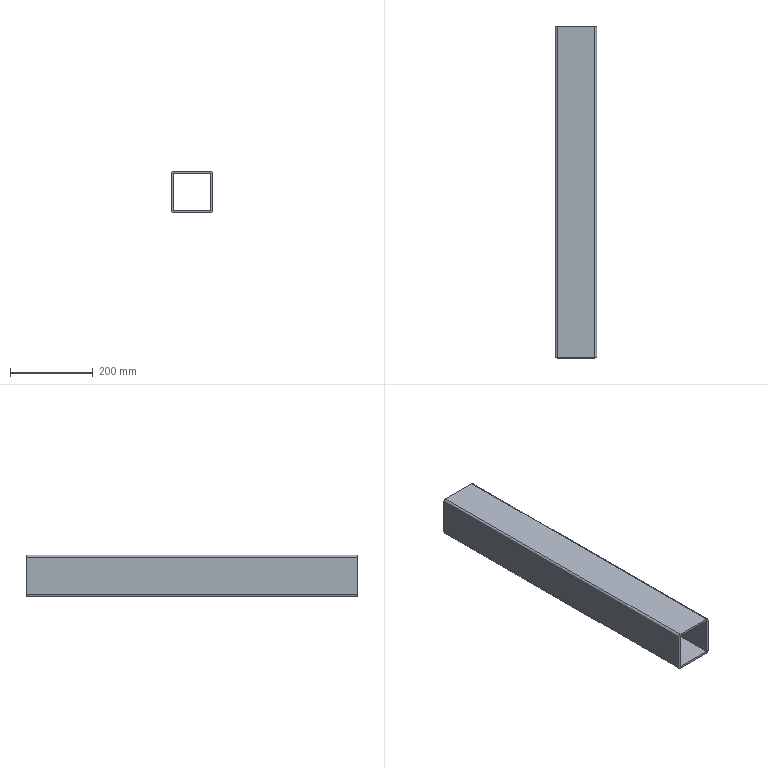Component | NX | TUBO | 1 solid | 14 faces | box 100 x 800 x 100 mm | volume 1502832 mm3 | plane 10 | cylinder 4 | commonest cylinder face diameters 10 x4
STEP:
#1=CARTESIAN_POINT('',(0.,0.,0.));
#2=DIRECTION('',(0.,0.,1.));
#3=DIRECTION('',(1.,0.,0.));
#4=AXIS2_PLACEMENT_3D('',#1,#2,#3);
#5=CARTESIAN_POINT('',(0.,65.2,795.));
#6=VERTEX_POINT('',#5);
#7=CARTESIAN_POINT('',(0.,65.2,705.));
#8=VERTEX_POINT('',#7);
#9=CARTESIAN_POINT('',(0.,65.2,795.));
#10=DIRECTION('',(0.,0.,-1.));
#11=VECTOR('',#10,1.);
#12=LINE('',#9,#11);
#13=CARTESIAN_POINT('',(0.,-734.8,795.));
#14=DIRECTION('',(1.,0.,0.));
#15=DIRECTION('',(0.,0.,-1.));
#16=AXIS2_PLACEMENT_3D('',#13,#14,#15);
#17=PLANE('',#16);
#18=CARTESIAN_POINT('',(0.,800.));
#19=DIRECTION('',(1.,0.));
#20=VECTOR('',#19,1.);
#21=LINE('',#18,#20);
#22=(GEOMETRIC_REPRESENTATION_CONTEXT(2)PARAMETRIC_REPRESENTATION_CONTEXT()REPRESENTATION_CONTEXT('',''));
#23=DEFINITIONAL_REPRESENTATION('',(#21),#22);
#24=PCURVE('',#17,#23);
#25=CARTESIAN_POINT('',(5.,65.2,705.));
#26=DIRECTION('',(0.,-1.,0.));
#27=DIRECTION('',(0.,0.,-1.));
#28=AXIS2_PLACEMENT_3D('',#25,#26,#27);
#29=PLANE('',#28);
#30=CARTESIAN_POINT('',(-90.,-5.));
#31=DIRECTION('',(1.,0.));
#32=VECTOR('',#31,1.);
#33=LINE('',#30,#32);
#34=(GEOMETRIC_REPRESENTATION_CONTEXT(2)PARAMETRIC_REPRESENTATION_CONTEXT()REPRESENTATION_CONTEXT('',''));
#35=DEFINITIONAL_REPRESENTATION('',(#33),#34);
#36=PCURVE('',#29,#35);
#37=SURFACE_CURVE('',#12,(#24,#36),.PCURVE_S1.);
#38=EDGE_CURVE('',#6,#8,#37,.T.);
#39=ORIENTED_EDGE('',*,*,#38,.T.);
#40=CARTESIAN_POINT('',(0.,-734.8,705.));
#41=VERTEX_POINT('',#40);
#42=CARTESIAN_POINT('',(0.,-734.8,705.));
#43=DIRECTION('',(0.,1.,0.));
#44=VECTOR('',#43,1.);
#45=LINE('',#42,#44);
#46=CARTESIAN_POINT('',(90.,0.));
#47=DIRECTION('',(0.,1.));
#48=VECTOR('',#47,1.);
#49=LINE('',#46,#48);
#50=(GEOMETRIC_REPRESENTATION_CONTEXT(2)PARAMETRIC_REPRESENTATION_CONTEXT()REPRESENTATION_CONTEXT('',''));
#51=DEFINITIONAL_REPRESENTATION('',(#49),#50);
#52=PCURVE('',#17,#51);
#53=CARTESIAN_POINT('',(5.,-734.8,705.));
#54=DIRECTION('',(0.,1.,0.));
#55=DIRECTION('',(0.,0.,1.));
#56=AXIS2_PLACEMENT_3D('',#53,#54,#55);
#57=CYLINDRICAL_SURFACE('',#56,5.);
#58=CARTESIAN_POINT('',(4.712,0.));
#59=DIRECTION('',(0.,1.));
#60=VECTOR('',#59,1.);
#61=LINE('',#58,#60);
#62=(GEOMETRIC_REPRESENTATION_CONTEXT(2)PARAMETRIC_REPRESENTATION_CONTEXT()REPRESENTATION_CONTEXT('',''));
#63=DEFINITIONAL_REPRESENTATION('',(#61),#62);
#64=PCURVE('',#57,#63);
#65=SURFACE_CURVE('',#45,(#52,#64),.PCURVE_S1.);
#66=EDGE_CURVE('',#41,#8,#65,.T.);
#67=ORIENTED_EDGE('',*,*,#66,.F.);
#68=CARTESIAN_POINT('',(0.,-734.8,795.));
#69=VERTEX_POINT('',#68);
#70=CARTESIAN_POINT('',(0.,-734.8,795.));
#71=DIRECTION('',(0.,0.,-1.));
#72=VECTOR('',#71,1.);
#73=LINE('',#70,#72);
#74=CARTESIAN_POINT('',(0.,0.));
#75=DIRECTION('',(1.,0.));
#76=VECTOR('',#75,1.);
#77=LINE('',#74,#76);
#78=(GEOMETRIC_REPRESENTATION_CONTEXT(2)PARAMETRIC_REPRESENTATION_CONTEXT()REPRESENTATION_CONTEXT('',''));
#79=DEFINITIONAL_REPRESENTATION('',(#77),#78);
#80=PCURVE('',#17,#79);
#81=CARTESIAN_POINT('',(5.,-734.8,705.));
#82=DIRECTION('',(0.,-1.,0.));
#83=DIRECTION('',(0.,0.,-1.));
#84=AXIS2_PLACEMENT_3D('',#81,#82,#83);
#85=PLANE('',#84);
#86=CARTESIAN_POINT('',(-90.,-5.));
#87=DIRECTION('',(1.,0.));
#88=VECTOR('',#87,1.);
#89=LINE('',#86,#88);
#90=(GEOMETRIC_REPRESENTATION_CONTEXT(2)PARAMETRIC_REPRESENTATION_CONTEXT()REPRESENTATION_CONTEXT('',''));
#91=DEFINITIONAL_REPRESENTATION('',(#89),#90);
#92=PCURVE('',#85,#91);
#93=SURFACE_CURVE('',#73,(#80,#92),.PCURVE_S1.);
#94=EDGE_CURVE('',#69,#41,#93,.T.);
#95=ORIENTED_EDGE('',*,*,#94,.F.);
#96=CARTESIAN_POINT('',(0.,-734.8,795.));
#97=DIRECTION('',(0.,1.,0.));
#98=VECTOR('',#97,1.);
#99=LINE('',#96,#98);
#100=CARTESIAN_POINT('',(0.,0.));
#101=DIRECTION('',(0.,1.));
#102=VECTOR('',#101,1.);
#103=LINE('',#100,#102);
#104=(GEOMETRIC_REPRESENTATION_CONTEXT(2)PARAMETRIC_REPRESENTATION_CONTEXT()REPRESENTATION_CONTEXT('',''));
#105=DEFINITIONAL_REPRESENTATION('',(#103),#104);
#106=PCURVE('',#17,#105);
#107=CARTESIAN_POINT('',(5.,-734.8,795.));
#108=DIRECTION('',(0.,1.,0.));
#109=DIRECTION('',(0.,0.,1.));
#110=AXIS2_PLACEMENT_3D('',#107,#108,#109);
#111=CYLINDRICAL_SURFACE('',#110,5.);
#112=CARTESIAN_POINT('',(4.712,0.));
#113=DIRECTION('',(0.,1.));
#114=VECTOR('',#113,1.);
#115=LINE('',#112,#114);
#116=(GEOMETRIC_REPRESENTATION_CONTEXT(2)PARAMETRIC_REPRESENTATION_CONTEXT()REPRESENTATION_CONTEXT('',''));
#117=DEFINITIONAL_REPRESENTATION('',(#115),#116);
#118=PCURVE('',#111,#117);
#119=SURFACE_CURVE('',#99,(#106,#118),.PCURVE_S1.);
#120=EDGE_CURVE('',#69,#6,#119,.T.);
#121=ORIENTED_EDGE('',*,*,#120,.T.);
#122=EDGE_LOOP('',(#39,#67,#95,#121));
#123=FACE_BOUND('',#122,.T.);
#124=ADVANCED_FACE('',(#123),#17,.F.);
#125=CARTESIAN_POINT('',(5.,65.2,700.));
#126=VERTEX_POINT('',#125);
#127=CARTESIAN_POINT('',(5.,65.2,705.));
#128=DIRECTION('',(0.,-1.,0.));
#129=DIRECTION('',(1.,0.,0.));
#130=AXIS2_PLACEMENT_3D('',#127,#128,#129);
#131=CIRCLE('',#130,5.);
#132=CARTESIAN_POINT('',(7.854,800.));
#133=DIRECTION('',(-1.,0.));
#134=VECTOR('',#133,1.);
#135=LINE('',#132,#134);
#136=(GEOMETRIC_REPRESENTATION_CONTEXT(2)PARAMETRIC_REPRESENTATION_CONTEXT()REPRESENTATION_CONTEXT('',''));
#137=DEFINITIONAL_REPRESENTATION('',(#135),#136);
#138=PCURVE('',#57,#137);
#139=CARTESIAN_POINT('',(0.,0.));
#140=DIRECTION('',(0.,1.));
#141=AXIS2_PLACEMENT_2D('',#139,#140);
#142=CIRCLE('',#141,5.);
#143=(GEOMETRIC_REPRESENTATION_CONTEXT(2)PARAMETRIC_REPRESENTATION_CONTEXT()REPRESENTATION_CONTEXT('',''));
#144=DEFINITIONAL_REPRESENTATION('',(#142),#143);
#145=PCURVE('',#29,#144);
#146=SURFACE_CURVE('',#131,(#138,#145),.PCURVE_S1.);
#147=EDGE_CURVE('',#8,#126,#146,.T.);
#148=ORIENTED_EDGE('',*,*,#147,.T.);
#149=CARTESIAN_POINT('',(5.,-734.8,700.));
#150=VERTEX_POINT('',#149);
#151=CARTESIAN_POINT('',(5.,-734.8,700.));
#152=DIRECTION('',(0.,1.,0.));
#153=VECTOR('',#152,1.);
#154=LINE('',#151,#153);
#155=CARTESIAN_POINT('',(3.142,0.));
#156=DIRECTION('',(0.,1.));
#157=VECTOR('',#156,1.);
#158=LINE('',#155,#157);
#159=(GEOMETRIC_REPRESENTATION_CONTEXT(2)PARAMETRIC_REPRESENTATION_CONTEXT()REPRESENTATION_CONTEXT('',''));
#160=DEFINITIONAL_REPRESENTATION('',(#158),#159);
#161=PCURVE('',#57,#160);
#162=CARTESIAN_POINT('',(5.,-734.8,700.));
#163=DIRECTION('',(-0.,0.,1.));
#164=DIRECTION('',(1.,0.,0.));
#165=AXIS2_PLACEMENT_3D('',#162,#163,#164);
#166=PLANE('',#165);
#167=CARTESIAN_POINT('',(-0.,0.));
#168=DIRECTION('',(0.,1.));
#169=VECTOR('',#168,1.);
#170=LINE('',#167,#169);
#171=(GEOMETRIC_REPRESENTATION_CONTEXT(2)PARAMETRIC_REPRESENTATION_CONTEXT()REPRESENTATION_CONTEXT('',''));
#172=DEFINITIONAL_REPRESENTATION('',(#170),#171);
#173=PCURVE('',#166,#172);
#174=SURFACE_CURVE('',#154,(#161,#173),.PCURVE_S1.);
#175=EDGE_CURVE('',#150,#126,#174,.T.);
#176=ORIENTED_EDGE('',*,*,#175,.F.);
#177=CARTESIAN_POINT('',(5.,-734.8,705.));
#178=DIRECTION('',(0.,-1.,0.));
#179=DIRECTION('',(1.,0.,0.));
#180=AXIS2_PLACEMENT_3D('',#177,#178,#179);
#181=CIRCLE('',#180,5.);
#182=CARTESIAN_POINT('',(7.854,0.));
#183=DIRECTION('',(-1.,0.));
#184=VECTOR('',#183,1.);
#185=LINE('',#182,#184);
#186=(GEOMETRIC_REPRESENTATION_CONTEXT(2)PARAMETRIC_REPRESENTATION_CONTEXT()REPRESENTATION_CONTEXT('',''));
#187=DEFINITIONAL_REPRESENTATION('',(#185),#186);
#188=PCURVE('',#57,#187);
#189=CARTESIAN_POINT('',(0.,0.));
#190=DIRECTION('',(0.,1.));
#191=AXIS2_PLACEMENT_2D('',#189,#190);
#192=CIRCLE('',#191,5.);
#193=(GEOMETRIC_REPRESENTATION_CONTEXT(2)PARAMETRIC_REPRESENTATION_CONTEXT()REPRESENTATION_CONTEXT('',''));
#194=DEFINITIONAL_REPRESENTATION('',(#192),#193);
#195=PCURVE('',#85,#194);
#196=SURFACE_CURVE('',#181,(#188,#195),.PCURVE_S1.);
#197=EDGE_CURVE('',#41,#150,#196,.T.);
#198=ORIENTED_EDGE('',*,*,#197,.F.);
#199=ORIENTED_EDGE('',*,*,#66,.T.);
#200=EDGE_LOOP('',(#148,#176,#198,#199));
#201=FACE_BOUND('',#200,.T.);
#202=ADVANCED_FACE('',(#201),#57,.T.);
#203=CARTESIAN_POINT('',(95.,65.2,700.));
#204=VERTEX_POINT('',#203);
#205=CARTESIAN_POINT('',(5.,65.2,700.));
#206=DIRECTION('',(1.,0.,0.));
#207=VECTOR('',#206,1.);
#208=LINE('',#205,#207);
#209=CARTESIAN_POINT('',(0.,800.));
#210=DIRECTION('',(1.,0.));
#211=VECTOR('',#210,1.);
#212=LINE('',#209,#211);
#213=(GEOMETRIC_REPRESENTATION_CONTEXT(2)PARAMETRIC_REPRESENTATION_CONTEXT()REPRESENTATION_CONTEXT('',''));
#214=DEFINITIONAL_REPRESENTATION('',(#212),#213);
#215=PCURVE('',#166,#214);
#216=CARTESIAN_POINT('',(5.,0.));
#217=DIRECTION('',(-0.,1.));
#218=VECTOR('',#217,1.);
#219=LINE('',#216,#218);
#220=(GEOMETRIC_REPRESENTATION_CONTEXT(2)PARAMETRIC_REPRESENTATION_CONTEXT()REPRESENTATION_CONTEXT('',''));
#221=DEFINITIONAL_REPRESENTATION('',(#219),#220);
#222=PCURVE('',#29,#221);
#223=SURFACE_CURVE('',#208,(#215,#222),.PCURVE_S1.);
#224=EDGE_CURVE('',#126,#204,#223,.T.);
#225=ORIENTED_EDGE('',*,*,#224,.T.);
#226=CARTESIAN_POINT('',(95.,-734.8,700.));
#227=VERTEX_POINT('',#226);
#228=CARTESIAN_POINT('',(95.,-734.8,700.));
#229=DIRECTION('',(0.,1.,0.));
#230=VECTOR('',#229,1.);
#231=LINE('',#228,#230);
#232=CARTESIAN_POINT('',(90.,0.));
#233=DIRECTION('',(0.,1.));
#234=VECTOR('',#233,1.);
#235=LINE('',#232,#234);
#236=(GEOMETRIC_REPRESENTATION_CONTEXT(2)PARAMETRIC_REPRESENTATION_CONTEXT()REPRESENTATION_CONTEXT('',''));
#237=DEFINITIONAL_REPRESENTATION('',(#235),#236);
#238=PCURVE('',#166,#237);
#239=CARTESIAN_POINT('',(95.,-734.8,705.));
#240=DIRECTION('',(0.,1.,0.));
#241=DIRECTION('',(0.,0.,1.));
#242=AXIS2_PLACEMENT_3D('',#239,#240,#241);
#243=CYLINDRICAL_SURFACE('',#242,5.);
#244=CARTESIAN_POINT('',(3.142,0.));
#245=DIRECTION('',(0.,1.));
#246=VECTOR('',#245,1.);
#247=LINE('',#244,#246);
#248=(GEOMETRIC_REPRESENTATION_CONTEXT(2)PARAMETRIC_REPRESENTATION_CONTEXT()REPRESENTATION_CONTEXT('',''));
#249=DEFINITIONAL_REPRESENTATION('',(#247),#248);
#250=PCURVE('',#243,#249);
#251=SURFACE_CURVE('',#231,(#238,#250),.PCURVE_S1.);
#252=EDGE_CURVE('',#227,#204,#251,.T.);
#253=ORIENTED_EDGE('',*,*,#252,.F.);
#254=CARTESIAN_POINT('',(5.,-734.8,700.));
#255=DIRECTION('',(1.,0.,0.));
#256=VECTOR('',#255,1.);
#257=LINE('',#254,#256);
#258=CARTESIAN_POINT('',(0.,0.));
#259=DIRECTION('',(1.,0.));
#260=VECTOR('',#259,1.);
#261=LINE('',#258,#260);
#262=(GEOMETRIC_REPRESENTATION_CONTEXT(2)PARAMETRIC_REPRESENTATION_CONTEXT()REPRESENTATION_CONTEXT('',''));
#263=DEFINITIONAL_REPRESENTATION('',(#261),#262);
#264=PCURVE('',#166,#263);
#265=CARTESIAN_POINT('',(5.,0.));
#266=DIRECTION('',(-0.,1.));
#267=VECTOR('',#266,1.);
#268=LINE('',#265,#267);
#269=(GEOMETRIC_REPRESENTATION_CONTEXT(2)PARAMETRIC_REPRESENTATION_CONTEXT()REPRESENTATION_CONTEXT('',''));
#270=DEFINITIONAL_REPRESENTATION('',(#268),#269);
#271=PCURVE('',#85,#270);
#272=SURFACE_CURVE('',#257,(#264,#271),.PCURVE_S1.);
#273=EDGE_CURVE('',#150,#227,#272,.T.);
#274=ORIENTED_EDGE('',*,*,#273,.F.);
#275=ORIENTED_EDGE('',*,*,#175,.T.);
#276=EDGE_LOOP('',(#225,#253,#274,#275));
#277=FACE_BOUND('',#276,.T.);
#278=ADVANCED_FACE('',(#277),#166,.F.);
#279=CARTESIAN_POINT('',(100.,65.2,705.));
#280=VERTEX_POINT('',#279);
#281=CARTESIAN_POINT('',(95.,65.2,705.));
#282=DIRECTION('',(0.,-1.,0.));
#283=DIRECTION('',(1.,0.,0.));
#284=AXIS2_PLACEMENT_3D('',#281,#282,#283);
#285=CIRCLE('',#284,5.);
#286=CARTESIAN_POINT('',(7.854,800.));
#287=DIRECTION('',(-1.,0.));
#288=VECTOR('',#287,1.);
#289=LINE('',#286,#288);
#290=(GEOMETRIC_REPRESENTATION_CONTEXT(2)PARAMETRIC_REPRESENTATION_CONTEXT()REPRESENTATION_CONTEXT('',''));
#291=DEFINITIONAL_REPRESENTATION('',(#289),#290);
#292=PCURVE('',#243,#291);
#293=CARTESIAN_POINT('',(0.,90.));
#294=DIRECTION('',(0.,1.));
#295=AXIS2_PLACEMENT_2D('',#293,#294);
#296=CIRCLE('',#295,5.);
#297=(GEOMETRIC_REPRESENTATION_CONTEXT(2)PARAMETRIC_REPRESENTATION_CONTEXT()REPRESENTATION_CONTEXT('',''));
#298=DEFINITIONAL_REPRESENTATION('',(#296),#297);
#299=PCURVE('',#29,#298);
#300=SURFACE_CURVE('',#285,(#292,#299),.PCURVE_S1.);
#301=EDGE_CURVE('',#204,#280,#300,.T.);
#302=ORIENTED_EDGE('',*,*,#301,.T.);
#303=CARTESIAN_POINT('',(100.,-734.8,705.));
#304=VERTEX_POINT('',#303);
#305=CARTESIAN_POINT('',(100.,-734.8,705.));
#306=DIRECTION('',(0.,1.,0.));
#307=VECTOR('',#306,1.);
#308=LINE('',#305,#307);
#309=CARTESIAN_POINT('',(1.571,0.));
#310=DIRECTION('',(0.,1.));
#311=VECTOR('',#310,1.);
#312=LINE('',#309,#311);
#313=(GEOMETRIC_REPRESENTATION_CONTEXT(2)PARAMETRIC_REPRESENTATION_CONTEXT()REPRESENTATION_CONTEXT('',''));
#314=DEFINITIONAL_REPRESENTATION('',(#312),#313);
#315=PCURVE('',#243,#314);
#316=CARTESIAN_POINT('',(100.,-734.8,705.));
#317=DIRECTION('',(-1.,0.,-0.));
#318=DIRECTION('',(-0.,0.,1.));
#319=AXIS2_PLACEMENT_3D('',#316,#317,#318);
#320=PLANE('',#319);
#321=CARTESIAN_POINT('',(0.,0.));
#322=DIRECTION('',(0.,1.));
#323=VECTOR('',#322,1.);
#324=LINE('',#321,#323);
#325=(GEOMETRIC_REPRESENTATION_CONTEXT(2)PARAMETRIC_REPRESENTATION_CONTEXT()REPRESENTATION_CONTEXT('',''));
#326=DEFINITIONAL_REPRESENTATION('',(#324),#325);
#327=PCURVE('',#320,#326);
#328=SURFACE_CURVE('',#308,(#315,#327),.PCURVE_S1.);
#329=EDGE_CURVE('',#304,#280,#328,.T.);
#330=ORIENTED_EDGE('',*,*,#329,.F.);
#331=CARTESIAN_POINT('',(95.,-734.8,705.));
#332=DIRECTION('',(0.,-1.,0.));
#333=DIRECTION('',(1.,0.,0.));
#334=AXIS2_PLACEMENT_3D('',#331,#332,#333);
#335=CIRCLE('',#334,5.);
#336=CARTESIAN_POINT('',(7.854,0.));
#337=DIRECTION('',(-1.,0.));
#338=VECTOR('',#337,1.);
#339=LINE('',#336,#338);
#340=(GEOMETRIC_REPRESENTATION_CONTEXT(2)PARAMETRIC_REPRESENTATION_CONTEXT()REPRESENTATION_CONTEXT('',''));
#341=DEFINITIONAL_REPRESENTATION('',(#339),#340);
#342=PCURVE('',#243,#341);
#343=CARTESIAN_POINT('',(0.,90.));
#344=DIRECTION('',(0.,1.));
#345=AXIS2_PLACEMENT_2D('',#343,#344);
#346=CIRCLE('',#345,5.);
#347=(GEOMETRIC_REPRESENTATION_CONTEXT(2)PARAMETRIC_REPRESENTATION_CONTEXT()REPRESENTATION_CONTEXT('',''));
#348=DEFINITIONAL_REPRESENTATION('',(#346),#347);
#349=PCURVE('',#85,#348);
#350=SURFACE_CURVE('',#335,(#342,#349),.PCURVE_S1.);
#351=EDGE_CURVE('',#227,#304,#350,.T.);
#352=ORIENTED_EDGE('',*,*,#351,.F.);
#353=ORIENTED_EDGE('',*,*,#252,.T.);
#354=EDGE_LOOP('',(#302,#330,#352,#353));
#355=FACE_BOUND('',#354,.T.);
#356=ADVANCED_FACE('',(#355),#243,.T.);
#357=CARTESIAN_POINT('',(100.,65.2,795.));
#358=VERTEX_POINT('',#357);
#359=CARTESIAN_POINT('',(100.,65.2,705.));
#360=DIRECTION('',(-0.,0.,1.));
#361=VECTOR('',#360,1.);
#362=LINE('',#359,#361);
#363=CARTESIAN_POINT('',(0.,800.));
#364=DIRECTION('',(1.,0.));
#365=VECTOR('',#364,1.);
#366=LINE('',#363,#365);
#367=(GEOMETRIC_REPRESENTATION_CONTEXT(2)PARAMETRIC_REPRESENTATION_CONTEXT()REPRESENTATION_CONTEXT('',''));
#368=DEFINITIONAL_REPRESENTATION('',(#366),#367);
#369=PCURVE('',#320,#368);
#370=CARTESIAN_POINT('',(0.,95.));
#371=DIRECTION('',(-1.,-0.));
#372=VECTOR('',#371,1.);
#373=LINE('',#370,#372);
#374=(GEOMETRIC_REPRESENTATION_CONTEXT(2)PARAMETRIC_REPRESENTATION_CONTEXT()REPRESENTATION_CONTEXT('',''));
#375=DEFINITIONAL_REPRESENTATION('',(#373),#374);
#376=PCURVE('',#29,#375);
#377=SURFACE_CURVE('',#362,(#369,#376),.PCURVE_S1.);
#378=EDGE_CURVE('',#280,#358,#377,.T.);
#379=ORIENTED_EDGE('',*,*,#378,.T.);
#380=CARTESIAN_POINT('',(100.,-734.8,795.));
#381=VERTEX_POINT('',#380);
#382=CARTESIAN_POINT('',(100.,-734.8,795.));
#383=DIRECTION('',(0.,1.,0.));
#384=VECTOR('',#383,1.);
#385=LINE('',#382,#384);
#386=CARTESIAN_POINT('',(90.,0.));
#387=DIRECTION('',(0.,1.));
#388=VECTOR('',#387,1.);
#389=LINE('',#386,#388);
#390=(GEOMETRIC_REPRESENTATION_CONTEXT(2)PARAMETRIC_REPRESENTATION_CONTEXT()REPRESENTATION_CONTEXT('',''));
#391=DEFINITIONAL_REPRESENTATION('',(#389),#390);
#392=PCURVE('',#320,#391);
#393=CARTESIAN_POINT('',(95.,-734.8,795.));
#394=DIRECTION('',(0.,1.,0.));
#395=DIRECTION('',(0.,0.,1.));
#396=AXIS2_PLACEMENT_3D('',#393,#394,#395);
#397=CYLINDRICAL_SURFACE('',#396,5.);
#398=CARTESIAN_POINT('',(1.571,0.));
#399=DIRECTION('',(0.,1.));
#400=VECTOR('',#399,1.);
#401=LINE('',#398,#400);
#402=(GEOMETRIC_REPRESENTATION_CONTEXT(2)PARAMETRIC_REPRESENTATION_CONTEXT()REPRESENTATION_CONTEXT('',''));
#403=DEFINITIONAL_REPRESENTATION('',(#401),#402);
#404=PCURVE('',#397,#403);
#405=SURFACE_CURVE('',#385,(#392,#404),.PCURVE_S1.);
#406=EDGE_CURVE('',#381,#358,#405,.T.);
#407=ORIENTED_EDGE('',*,*,#406,.F.);
#408=CARTESIAN_POINT('',(100.,-734.8,705.));
#409=DIRECTION('',(-0.,0.,1.));
#410=VECTOR('',#409,1.);
#411=LINE('',#408,#410);
#412=CARTESIAN_POINT('',(0.,0.));
#413=DIRECTION('',(1.,0.));
#414=VECTOR('',#413,1.);
#415=LINE('',#412,#414);
#416=(GEOMETRIC_REPRESENTATION_CONTEXT(2)PARAMETRIC_REPRESENTATION_CONTEXT()REPRESENTATION_CONTEXT('',''));
#417=DEFINITIONAL_REPRESENTATION('',(#415),#416);
#418=PCURVE('',#320,#417);
#419=CARTESIAN_POINT('',(0.,95.));
#420=DIRECTION('',(-1.,-0.));
#421=VECTOR('',#420,1.);
#422=LINE('',#419,#421);
#423=(GEOMETRIC_REPRESENTATION_CONTEXT(2)PARAMETRIC_REPRESENTATION_CONTEXT()REPRESENTATION_CONTEXT('',''));
#424=DEFINITIONAL_REPRESENTATION('',(#422),#423);
#425=PCURVE('',#85,#424);
#426=SURFACE_CURVE('',#411,(#418,#425),.PCURVE_S1.);
#427=EDGE_CURVE('',#304,#381,#426,.T.);
#428=ORIENTED_EDGE('',*,*,#427,.F.);
#429=ORIENTED_EDGE('',*,*,#329,.T.);
#430=EDGE_LOOP('',(#379,#407,#428,#429));
#431=FACE_BOUND('',#430,.T.);
#432=ADVANCED_FACE('',(#431),#320,.F.);
#433=CARTESIAN_POINT('',(95.,65.2,800.));
#434=VERTEX_POINT('',#433);
#435=CARTESIAN_POINT('',(95.,65.2,795.));
#436=DIRECTION('',(0.,-1.,0.));
#437=DIRECTION('',(1.,0.,0.));
#438=AXIS2_PLACEMENT_3D('',#435,#436,#437);
#439=CIRCLE('',#438,5.);
#440=CARTESIAN_POINT('',(1.571,800.));
#441=DIRECTION('',(-1.,0.));
#442=VECTOR('',#441,1.);
#443=LINE('',#440,#442);
#444=(GEOMETRIC_REPRESENTATION_CONTEXT(2)PARAMETRIC_REPRESENTATION_CONTEXT()REPRESENTATION_CONTEXT('',''));
#445=DEFINITIONAL_REPRESENTATION('',(#443),#444);
#446=PCURVE('',#397,#445);
#447=CARTESIAN_POINT('',(-90.,90.));
#448=DIRECTION('',(0.,1.));
#449=AXIS2_PLACEMENT_2D('',#447,#448);
#450=CIRCLE('',#449,5.);
#451=(GEOMETRIC_REPRESENTATION_CONTEXT(2)PARAMETRIC_REPRESENTATION_CONTEXT()REPRESENTATION_CONTEXT('',''));
#452=DEFINITIONAL_REPRESENTATION('',(#450),#451);
#453=PCURVE('',#29,#452);
#454=SURFACE_CURVE('',#439,(#446,#453),.PCURVE_S1.);
#455=EDGE_CURVE('',#358,#434,#454,.T.);
#456=ORIENTED_EDGE('',*,*,#455,.T.);
#457=CARTESIAN_POINT('',(95.,-734.8,800.));
#458=VERTEX_POINT('',#457);
#459=CARTESIAN_POINT('',(95.,-734.8,800.));
#460=DIRECTION('',(0.,1.,0.));
#461=VECTOR('',#460,1.);
#462=LINE('',#459,#461);
#463=CARTESIAN_POINT('',(0.,0.));
#464=DIRECTION('',(0.,1.));
#465=VECTOR('',#464,1.);
#466=LINE('',#463,#465);
#467=(GEOMETRIC_REPRESENTATION_CONTEXT(2)PARAMETRIC_REPRESENTATION_CONTEXT()REPRESENTATION_CONTEXT('',''));
#468=DEFINITIONAL_REPRESENTATION('',(#466),#467);
#469=PCURVE('',#397,#468);
#470=CARTESIAN_POINT('',(95.,-734.8,800.));
#471=DIRECTION('',(0.,0.,-1.));
#472=DIRECTION('',(-1.,0.,-0.));
#473=AXIS2_PLACEMENT_3D('',#470,#471,#472);
#474=PLANE('',#473);
#475=CARTESIAN_POINT('',(0.,0.));
#476=DIRECTION('',(0.,1.));
#477=VECTOR('',#476,1.);
#478=LINE('',#475,#477);
#479=(GEOMETRIC_REPRESENTATION_CONTEXT(2)PARAMETRIC_REPRESENTATION_CONTEXT()REPRESENTATION_CONTEXT('',''));
#480=DEFINITIONAL_REPRESENTATION('',(#478),#479);
#481=PCURVE('',#474,#480);
#482=SURFACE_CURVE('',#462,(#469,#481),.PCURVE_S1.);
#483=EDGE_CURVE('',#458,#434,#482,.T.);
#484=ORIENTED_EDGE('',*,*,#483,.F.);
#485=CARTESIAN_POINT('',(95.,-734.8,795.));
#486=DIRECTION('',(0.,-1.,0.));
#487=DIRECTION('',(1.,0.,0.));
#488=AXIS2_PLACEMENT_3D('',#485,#486,#487);
#489=CIRCLE('',#488,5.);
#490=CARTESIAN_POINT('',(1.571,0.));
#491=DIRECTION('',(-1.,0.));
#492=VECTOR('',#491,1.);
#493=LINE('',#490,#492);
#494=(GEOMETRIC_REPRESENTATION_CONTEXT(2)PARAMETRIC_REPRESENTATION_CONTEXT()REPRESENTATION_CONTEXT('',''));
#495=DEFINITIONAL_REPRESENTATION('',(#493),#494);
#496=PCURVE('',#397,#495);
#497=CARTESIAN_POINT('',(-90.,90.));
#498=DIRECTION('',(0.,1.));
#499=AXIS2_PLACEMENT_2D('',#497,#498);
#500=CIRCLE('',#499,5.);
#501=(GEOMETRIC_REPRESENTATION_CONTEXT(2)PARAMETRIC_REPRESENTATION_CONTEXT()REPRESENTATION_CONTEXT('',''));
#502=DEFINITIONAL_REPRESENTATION('',(#500),#501);
#503=PCURVE('',#85,#502);
#504=SURFACE_CURVE('',#489,(#496,#503),.PCURVE_S1.);
#505=EDGE_CURVE('',#381,#458,#504,.T.);
#506=ORIENTED_EDGE('',*,*,#505,.F.);
#507=ORIENTED_EDGE('',*,*,#406,.T.);
#508=EDGE_LOOP('',(#456,#484,#506,#507));
#509=FACE_BOUND('',#508,.T.);
#510=ADVANCED_FACE('',(#509),#397,.T.);
#511=CARTESIAN_POINT('',(5.,65.2,800.));
#512=VERTEX_POINT('',#511);
#513=CARTESIAN_POINT('',(95.,65.2,800.));
#514=DIRECTION('',(-1.,0.,-0.));
#515=VECTOR('',#514,1.);
#516=LINE('',#513,#515);
#517=CARTESIAN_POINT('',(0.,800.));
#518=DIRECTION('',(1.,0.));
#519=VECTOR('',#518,1.);
#520=LINE('',#517,#519);
#521=(GEOMETRIC_REPRESENTATION_CONTEXT(2)PARAMETRIC_REPRESENTATION_CONTEXT()REPRESENTATION_CONTEXT('',''));
#522=DEFINITIONAL_REPRESENTATION('',(#520),#521);
#523=PCURVE('',#474,#522);
#524=CARTESIAN_POINT('',(-95.,90.));
#525=DIRECTION('',(0.,-1.));
#526=VECTOR('',#525,1.);
#527=LINE('',#524,#526);
#528=(GEOMETRIC_REPRESENTATION_CONTEXT(2)PARAMETRIC_REPRESENTATION_CONTEXT()REPRESENTATION_CONTEXT('',''));
#529=DEFINITIONAL_REPRESENTATION('',(#527),#528);
#530=PCURVE('',#29,#529);
#531=SURFACE_CURVE('',#516,(#523,#530),.PCURVE_S1.);
#532=EDGE_CURVE('',#434,#512,#531,.T.);
#533=ORIENTED_EDGE('',*,*,#532,.T.);
#534=CARTESIAN_POINT('',(5.,-734.8,800.));
#535=VERTEX_POINT('',#534);
#536=CARTESIAN_POINT('',(5.,-734.8,800.));
#537=DIRECTION('',(0.,1.,0.));
#538=VECTOR('',#537,1.);
#539=LINE('',#536,#538);
#540=CARTESIAN_POINT('',(90.,0.));
#541=DIRECTION('',(0.,1.));
#542=VECTOR('',#541,1.);
#543=LINE('',#540,#542);
#544=(GEOMETRIC_REPRESENTATION_CONTEXT(2)PARAMETRIC_REPRESENTATION_CONTEXT()REPRESENTATION_CONTEXT('',''));
#545=DEFINITIONAL_REPRESENTATION('',(#543),#544);
#546=PCURVE('',#474,#545);
#547=CARTESIAN_POINT('',(6.283,0.));
#548=DIRECTION('',(0.,1.));
#549=VECTOR('',#548,1.);
#550=LINE('',#547,#549);
#551=(GEOMETRIC_REPRESENTATION_CONTEXT(2)PARAMETRIC_REPRESENTATION_CONTEXT()REPRESENTATION_CONTEXT('',''));
#552=DEFINITIONAL_REPRESENTATION('',(#550),#551);
#553=PCURVE('',#111,#552);
#554=SURFACE_CURVE('',#539,(#546,#553),.PCURVE_S1.);
#555=EDGE_CURVE('',#535,#512,#554,.T.);
#556=ORIENTED_EDGE('',*,*,#555,.F.);
#557=CARTESIAN_POINT('',(95.,-734.8,800.));
#558=DIRECTION('',(-1.,0.,-0.));
#559=VECTOR('',#558,1.);
#560=LINE('',#557,#559);
#561=CARTESIAN_POINT('',(0.,0.));
#562=DIRECTION('',(1.,0.));
#563=VECTOR('',#562,1.);
#564=LINE('',#561,#563);
#565=(GEOMETRIC_REPRESENTATION_CONTEXT(2)PARAMETRIC_REPRESENTATION_CONTEXT()REPRESENTATION_CONTEXT('',''));
#566=DEFINITIONAL_REPRESENTATION('',(#564),#565);
#567=PCURVE('',#474,#566);
#568=CARTESIAN_POINT('',(-95.,90.));
#569=DIRECTION('',(0.,-1.));
#570=VECTOR('',#569,1.);
#571=LINE('',#568,#570);
#572=(GEOMETRIC_REPRESENTATION_CONTEXT(2)PARAMETRIC_REPRESENTATION_CONTEXT()REPRESENTATION_CONTEXT('',''));
#573=DEFINITIONAL_REPRESENTATION('',(#571),#572);
#574=PCURVE('',#85,#573);
#575=SURFACE_CURVE('',#560,(#567,#574),.PCURVE_S1.);
#576=EDGE_CURVE('',#458,#535,#575,.T.);
#577=ORIENTED_EDGE('',*,*,#576,.F.);
#578=ORIENTED_EDGE('',*,*,#483,.T.);
#579=EDGE_LOOP('',(#533,#556,#577,#578));
#580=FACE_BOUND('',#579,.T.);
#581=ADVANCED_FACE('',(#580),#474,.F.);
#582=CARTESIAN_POINT('',(5.,65.2,795.));
#583=DIRECTION('',(0.,-1.,0.));
#584=DIRECTION('',(1.,0.,0.));
#585=AXIS2_PLACEMENT_3D('',#582,#583,#584);
#586=CIRCLE('',#585,5.);
#587=CARTESIAN_POINT('',(7.854,800.));
#588=DIRECTION('',(-1.,0.));
#589=VECTOR('',#588,1.);
#590=LINE('',#587,#589);
#591=(GEOMETRIC_REPRESENTATION_CONTEXT(2)PARAMETRIC_REPRESENTATION_CONTEXT()REPRESENTATION_CONTEXT('',''));
#592=DEFINITIONAL_REPRESENTATION('',(#590),#591);
#593=PCURVE('',#111,#592);
#594=CARTESIAN_POINT('',(-90.,0.));
#595=DIRECTION('',(0.,1.));
#596=AXIS2_PLACEMENT_2D('',#594,#595);
#597=CIRCLE('',#596,5.);
#598=(GEOMETRIC_REPRESENTATION_CONTEXT(2)PARAMETRIC_REPRESENTATION_CONTEXT()REPRESENTATION_CONTEXT('',''));
#599=DEFINITIONAL_REPRESENTATION('',(#597),#598);
#600=PCURVE('',#29,#599);
#601=SURFACE_CURVE('',#586,(#593,#600),.PCURVE_S1.);
#602=EDGE_CURVE('',#512,#6,#601,.T.);
#603=ORIENTED_EDGE('',*,*,#602,.T.);
#604=ORIENTED_EDGE('',*,*,#120,.F.);
#605=CARTESIAN_POINT('',(5.,-734.8,795.));
#606=DIRECTION('',(0.,-1.,0.));
#607=DIRECTION('',(1.,0.,0.));
#608=AXIS2_PLACEMENT_3D('',#605,#606,#607);
#609=CIRCLE('',#608,5.);
#610=CARTESIAN_POINT('',(7.854,0.));
#611=DIRECTION('',(-1.,0.));
#612=VECTOR('',#611,1.);
#613=LINE('',#610,#612);
#614=(GEOMETRIC_REPRESENTATION_CONTEXT(2)PARAMETRIC_REPRESENTATION_CONTEXT()REPRESENTATION_CONTEXT('',''));
#615=DEFINITIONAL_REPRESENTATION('',(#613),#614);
#616=PCURVE('',#111,#615);
#617=CARTESIAN_POINT('',(-90.,0.));
#618=DIRECTION('',(0.,1.));
#619=AXIS2_PLACEMENT_2D('',#617,#618);
#620=CIRCLE('',#619,5.);
#621=(GEOMETRIC_REPRESENTATION_CONTEXT(2)PARAMETRIC_REPRESENTATION_CONTEXT()REPRESENTATION_CONTEXT('',''));
#622=DEFINITIONAL_REPRESENTATION('',(#620),#621);
#623=PCURVE('',#85,#622);
#624=SURFACE_CURVE('',#609,(#616,#623),.PCURVE_S1.);
#625=EDGE_CURVE('',#535,#69,#624,.T.);
#626=ORIENTED_EDGE('',*,*,#625,.F.);
#627=ORIENTED_EDGE('',*,*,#555,.T.);
#628=EDGE_LOOP('',(#603,#604,#626,#627));
#629=FACE_BOUND('',#628,.T.);
#630=ADVANCED_FACE('',(#629),#111,.T.);
#631=CARTESIAN_POINT('',(5.,-734.8,795.));
#632=VERTEX_POINT('',#631);
#633=CARTESIAN_POINT('',(5.,-734.8,705.));
#634=VERTEX_POINT('',#633);
#635=CARTESIAN_POINT('',(5.,-734.8,795.));
#636=DIRECTION('',(0.,0.,-1.));
#637=VECTOR('',#636,1.);
#638=LINE('',#635,#637);
#639=CARTESIAN_POINT('',(-90.,0.));
#640=DIRECTION('',(1.,0.));
#641=VECTOR('',#640,1.);
#642=LINE('',#639,#641);
#643=(GEOMETRIC_REPRESENTATION_CONTEXT(2)PARAMETRIC_REPRESENTATION_CONTEXT()REPRESENTATION_CONTEXT('',''));
#644=DEFINITIONAL_REPRESENTATION('',(#642),#643);
#645=PCURVE('',#85,#644);
#646=CARTESIAN_POINT('',(5.,-734.8,795.));
#647=DIRECTION('',(1.,0.,0.));
#648=DIRECTION('',(0.,0.,-1.));
#649=AXIS2_PLACEMENT_3D('',#646,#647,#648);
#650=PLANE('',#649);
#651=CARTESIAN_POINT('',(0.,0.));
#652=DIRECTION('',(1.,0.));
#653=VECTOR('',#652,1.);
#654=LINE('',#651,#653);
#655=(GEOMETRIC_REPRESENTATION_CONTEXT(2)PARAMETRIC_REPRESENTATION_CONTEXT()REPRESENTATION_CONTEXT('',''));
#656=DEFINITIONAL_REPRESENTATION('',(#654),#655);
#657=PCURVE('',#650,#656);
#658=SURFACE_CURVE('',#638,(#645,#657),.PCURVE_S1.);
#659=EDGE_CURVE('',#632,#634,#658,.T.);
#660=ORIENTED_EDGE('',*,*,#659,.F.);
#661=CARTESIAN_POINT('',(95.,-734.8,795.));
#662=VERTEX_POINT('',#661);
#663=CARTESIAN_POINT('',(95.,-734.8,795.));
#664=DIRECTION('',(-1.,0.,-0.));
#665=VECTOR('',#664,1.);
#666=LINE('',#663,#665);
#667=CARTESIAN_POINT('',(-90.,90.));
#668=DIRECTION('',(0.,-1.));
#669=VECTOR('',#668,1.);
#670=LINE('',#667,#669);
#671=(GEOMETRIC_REPRESENTATION_CONTEXT(2)PARAMETRIC_REPRESENTATION_CONTEXT()REPRESENTATION_CONTEXT('',''));
#672=DEFINITIONAL_REPRESENTATION('',(#670),#671);
#673=PCURVE('',#85,#672);
#674=CARTESIAN_POINT('',(95.,-734.8,795.));
#675=DIRECTION('',(0.,0.,-1.));
#676=DIRECTION('',(-1.,0.,-0.));
#677=AXIS2_PLACEMENT_3D('',#674,#675,#676);
#678=PLANE('',#677);
#679=CARTESIAN_POINT('',(0.,0.));
#680=DIRECTION('',(1.,0.));
#681=VECTOR('',#680,1.);
#682=LINE('',#679,#681);
#683=(GEOMETRIC_REPRESENTATION_CONTEXT(2)PARAMETRIC_REPRESENTATION_CONTEXT()REPRESENTATION_CONTEXT('',''));
#684=DEFINITIONAL_REPRESENTATION('',(#682),#683);
#685=PCURVE('',#678,#684);
#686=SURFACE_CURVE('',#666,(#673,#685),.PCURVE_S1.);
#687=EDGE_CURVE('',#662,#632,#686,.T.);
#688=ORIENTED_EDGE('',*,*,#687,.F.);
#689=CARTESIAN_POINT('',(95.,-734.8,705.));
#690=VERTEX_POINT('',#689);
#691=CARTESIAN_POINT('',(95.,-734.8,705.));
#692=DIRECTION('',(-0.,0.,1.));
#693=VECTOR('',#692,1.);
#694=LINE('',#691,#693);
#695=CARTESIAN_POINT('',(0.,90.));
#696=DIRECTION('',(-1.,-0.));
#697=VECTOR('',#696,1.);
#698=LINE('',#695,#697);
#699=(GEOMETRIC_REPRESENTATION_CONTEXT(2)PARAMETRIC_REPRESENTATION_CONTEXT()REPRESENTATION_CONTEXT('',''));
#700=DEFINITIONAL_REPRESENTATION('',(#698),#699);
#701=PCURVE('',#85,#700);
#702=CARTESIAN_POINT('',(95.,-734.8,705.));
#703=DIRECTION('',(-1.,0.,-0.));
#704=DIRECTION('',(-0.,0.,1.));
#705=AXIS2_PLACEMENT_3D('',#702,#703,#704);
#706=PLANE('',#705);
#707=CARTESIAN_POINT('',(0.,0.));
#708=DIRECTION('',(1.,0.));
#709=VECTOR('',#708,1.);
#710=LINE('',#707,#709);
#711=(GEOMETRIC_REPRESENTATION_CONTEXT(2)PARAMETRIC_REPRESENTATION_CONTEXT()REPRESENTATION_CONTEXT('',''));
#712=DEFINITIONAL_REPRESENTATION('',(#710),#711);
#713=PCURVE('',#706,#712);
#714=SURFACE_CURVE('',#694,(#701,#713),.PCURVE_S1.);
#715=EDGE_CURVE('',#690,#662,#714,.T.);
#716=ORIENTED_EDGE('',*,*,#715,.F.);
#717=CARTESIAN_POINT('',(5.,-734.8,705.));
#718=DIRECTION('',(1.,0.,0.));
#719=VECTOR('',#718,1.);
#720=LINE('',#717,#719);
#721=CARTESIAN_POINT('',(0.,0.));
#722=DIRECTION('',(-0.,1.));
#723=VECTOR('',#722,1.);
#724=LINE('',#721,#723);
#725=(GEOMETRIC_REPRESENTATION_CONTEXT(2)PARAMETRIC_REPRESENTATION_CONTEXT()REPRESENTATION_CONTEXT('',''));
#726=DEFINITIONAL_REPRESENTATION('',(#724),#725);
#727=PCURVE('',#85,#726);
#728=CARTESIAN_POINT('',(5.,-734.8,705.));
#729=DIRECTION('',(-0.,0.,1.));
#730=DIRECTION('',(1.,0.,0.));
#731=AXIS2_PLACEMENT_3D('',#728,#729,#730);
#732=PLANE('',#731);
#733=CARTESIAN_POINT('',(0.,0.));
#734=DIRECTION('',(1.,0.));
#735=VECTOR('',#734,1.);
#736=LINE('',#733,#735);
#737=(GEOMETRIC_REPRESENTATION_CONTEXT(2)PARAMETRIC_REPRESENTATION_CONTEXT()REPRESENTATION_CONTEXT('',''));
#738=DEFINITIONAL_REPRESENTATION('',(#736),#737);
#739=PCURVE('',#732,#738);
#740=SURFACE_CURVE('',#720,(#727,#739),.PCURVE_S1.);
#741=EDGE_CURVE('',#634,#690,#740,.T.);
#742=ORIENTED_EDGE('',*,*,#741,.F.);
#743=EDGE_LOOP('',(#660,#688,#716,#742));
#744=FACE_BOUND('',#743,.T.);
#745=ORIENTED_EDGE('',*,*,#94,.T.);
#746=ORIENTED_EDGE('',*,*,#197,.T.);
#747=ORIENTED_EDGE('',*,*,#273,.T.);
#748=ORIENTED_EDGE('',*,*,#351,.T.);
#749=ORIENTED_EDGE('',*,*,#427,.T.);
#750=ORIENTED_EDGE('',*,*,#505,.T.);
#751=ORIENTED_EDGE('',*,*,#576,.T.);
#752=ORIENTED_EDGE('',*,*,#625,.T.);
#753=EDGE_LOOP('',(#745,#746,#747,#748,#749,#750,#751,#752));
#754=FACE_BOUND('',#753,.T.);
#755=ADVANCED_FACE('',(#744,#754),#85,.T.);
#756=CARTESIAN_POINT('',(95.,65.2,795.));
#757=VERTEX_POINT('',#756);
#758=CARTESIAN_POINT('',(5.,65.2,795.));
#759=VERTEX_POINT('',#758);
#760=CARTESIAN_POINT('',(95.,65.2,795.));
#761=DIRECTION('',(-1.,0.,-0.));
#762=VECTOR('',#761,1.);
#763=LINE('',#760,#762);
#764=CARTESIAN_POINT('',(-90.,90.));
#765=DIRECTION('',(0.,-1.));
#766=VECTOR('',#765,1.);
#767=LINE('',#764,#766);
#768=(GEOMETRIC_REPRESENTATION_CONTEXT(2)PARAMETRIC_REPRESENTATION_CONTEXT()REPRESENTATION_CONTEXT('',''));
#769=DEFINITIONAL_REPRESENTATION('',(#767),#768);
#770=PCURVE('',#29,#769);
#771=CARTESIAN_POINT('',(0.,800.));
#772=DIRECTION('',(1.,0.));
#773=VECTOR('',#772,1.);
#774=LINE('',#771,#773);
#775=(GEOMETRIC_REPRESENTATION_CONTEXT(2)PARAMETRIC_REPRESENTATION_CONTEXT()REPRESENTATION_CONTEXT('',''));
#776=DEFINITIONAL_REPRESENTATION('',(#774),#775);
#777=PCURVE('',#678,#776);
#778=SURFACE_CURVE('',#763,(#770,#777),.PCURVE_S1.);
#779=EDGE_CURVE('',#757,#759,#778,.T.);
#780=ORIENTED_EDGE('',*,*,#779,.T.);
#781=CARTESIAN_POINT('',(5.,65.2,705.));
#782=VERTEX_POINT('',#781);
#783=CARTESIAN_POINT('',(5.,65.2,795.));
#784=DIRECTION('',(0.,0.,-1.));
#785=VECTOR('',#784,1.);
#786=LINE('',#783,#785);
#787=CARTESIAN_POINT('',(-90.,0.));
#788=DIRECTION('',(1.,0.));
#789=VECTOR('',#788,1.);
#790=LINE('',#787,#789);
#791=(GEOMETRIC_REPRESENTATION_CONTEXT(2)PARAMETRIC_REPRESENTATION_CONTEXT()REPRESENTATION_CONTEXT('',''));
#792=DEFINITIONAL_REPRESENTATION('',(#790),#791);
#793=PCURVE('',#29,#792);
#794=CARTESIAN_POINT('',(0.,800.));
#795=DIRECTION('',(1.,0.));
#796=VECTOR('',#795,1.);
#797=LINE('',#794,#796);
#798=(GEOMETRIC_REPRESENTATION_CONTEXT(2)PARAMETRIC_REPRESENTATION_CONTEXT()REPRESENTATION_CONTEXT('',''));
#799=DEFINITIONAL_REPRESENTATION('',(#797),#798);
#800=PCURVE('',#650,#799);
#801=SURFACE_CURVE('',#786,(#793,#800),.PCURVE_S1.);
#802=EDGE_CURVE('',#759,#782,#801,.T.);
#803=ORIENTED_EDGE('',*,*,#802,.T.);
#804=CARTESIAN_POINT('',(95.,65.2,705.));
#805=VERTEX_POINT('',#804);
#806=CARTESIAN_POINT('',(5.,65.2,705.));
#807=DIRECTION('',(1.,0.,0.));
#808=VECTOR('',#807,1.);
#809=LINE('',#806,#808);
#810=CARTESIAN_POINT('',(0.,0.));
#811=DIRECTION('',(-0.,1.));
#812=VECTOR('',#811,1.);
#813=LINE('',#810,#812);
#814=(GEOMETRIC_REPRESENTATION_CONTEXT(2)PARAMETRIC_REPRESENTATION_CONTEXT()REPRESENTATION_CONTEXT('',''));
#815=DEFINITIONAL_REPRESENTATION('',(#813),#814);
#816=PCURVE('',#29,#815);
#817=CARTESIAN_POINT('',(0.,800.));
#818=DIRECTION('',(1.,0.));
#819=VECTOR('',#818,1.);
#820=LINE('',#817,#819);
#821=(GEOMETRIC_REPRESENTATION_CONTEXT(2)PARAMETRIC_REPRESENTATION_CONTEXT()REPRESENTATION_CONTEXT('',''));
#822=DEFINITIONAL_REPRESENTATION('',(#820),#821);
#823=PCURVE('',#732,#822);
#824=SURFACE_CURVE('',#809,(#816,#823),.PCURVE_S1.);
#825=EDGE_CURVE('',#782,#805,#824,.T.);
#826=ORIENTED_EDGE('',*,*,#825,.T.);
#827=CARTESIAN_POINT('',(95.,65.2,705.));
#828=DIRECTION('',(-0.,0.,1.));
#829=VECTOR('',#828,1.);
#830=LINE('',#827,#829);
#831=CARTESIAN_POINT('',(0.,90.));
#832=DIRECTION('',(-1.,-0.));
#833=VECTOR('',#832,1.);
#834=LINE('',#831,#833);
#835=(GEOMETRIC_REPRESENTATION_CONTEXT(2)PARAMETRIC_REPRESENTATION_CONTEXT()REPRESENTATION_CONTEXT('',''));
#836=DEFINITIONAL_REPRESENTATION('',(#834),#835);
#837=PCURVE('',#29,#836);
#838=CARTESIAN_POINT('',(0.,800.));
#839=DIRECTION('',(1.,0.));
#840=VECTOR('',#839,1.);
#841=LINE('',#838,#840);
#842=(GEOMETRIC_REPRESENTATION_CONTEXT(2)PARAMETRIC_REPRESENTATION_CONTEXT()REPRESENTATION_CONTEXT('',''));
#843=DEFINITIONAL_REPRESENTATION('',(#841),#842);
#844=PCURVE('',#706,#843);
#845=SURFACE_CURVE('',#830,(#837,#844),.PCURVE_S1.);
#846=EDGE_CURVE('',#805,#757,#845,.T.);
#847=ORIENTED_EDGE('',*,*,#846,.T.);
#848=EDGE_LOOP('',(#780,#803,#826,#847));
#849=FACE_BOUND('',#848,.T.);
#850=ORIENTED_EDGE('',*,*,#38,.F.);
#851=ORIENTED_EDGE('',*,*,#602,.F.);
#852=ORIENTED_EDGE('',*,*,#532,.F.);
#853=ORIENTED_EDGE('',*,*,#455,.F.);
#854=ORIENTED_EDGE('',*,*,#378,.F.);
#855=ORIENTED_EDGE('',*,*,#301,.F.);
#856=ORIENTED_EDGE('',*,*,#224,.F.);
#857=ORIENTED_EDGE('',*,*,#147,.F.);
#858=EDGE_LOOP('',(#850,#851,#852,#853,#854,#855,#856,#857));
#859=FACE_BOUND('',#858,.T.);
#860=ADVANCED_FACE('',(#849,#859),#29,.F.);
#861=ORIENTED_EDGE('',*,*,#802,.F.);
#862=CARTESIAN_POINT('',(5.,-734.8,795.));
#863=DIRECTION('',(0.,1.,0.));
#864=VECTOR('',#863,1.);
#865=LINE('',#862,#864);
#866=CARTESIAN_POINT('',(0.,0.));
#867=DIRECTION('',(0.,1.));
#868=VECTOR('',#867,1.);
#869=LINE('',#866,#868);
#870=(GEOMETRIC_REPRESENTATION_CONTEXT(2)PARAMETRIC_REPRESENTATION_CONTEXT()REPRESENTATION_CONTEXT('',''));
#871=DEFINITIONAL_REPRESENTATION('',(#869),#870);
#872=PCURVE('',#650,#871);
#873=CARTESIAN_POINT('',(90.,0.));
#874=DIRECTION('',(0.,1.));
#875=VECTOR('',#874,1.);
#876=LINE('',#873,#875);
#877=(GEOMETRIC_REPRESENTATION_CONTEXT(2)PARAMETRIC_REPRESENTATION_CONTEXT()REPRESENTATION_CONTEXT('',''));
#878=DEFINITIONAL_REPRESENTATION('',(#876),#877);
#879=PCURVE('',#678,#878);
#880=SURFACE_CURVE('',#865,(#872,#879),.PCURVE_S1.);
#881=EDGE_CURVE('',#632,#759,#880,.T.);
#882=ORIENTED_EDGE('',*,*,#881,.F.);
#883=ORIENTED_EDGE('',*,*,#659,.T.);
#884=CARTESIAN_POINT('',(5.,-734.8,705.));
#885=DIRECTION('',(0.,1.,0.));
#886=VECTOR('',#885,1.);
#887=LINE('',#884,#886);
#888=CARTESIAN_POINT('',(90.,0.));
#889=DIRECTION('',(0.,1.));
#890=VECTOR('',#889,1.);
#891=LINE('',#888,#890);
#892=(GEOMETRIC_REPRESENTATION_CONTEXT(2)PARAMETRIC_REPRESENTATION_CONTEXT()REPRESENTATION_CONTEXT('',''));
#893=DEFINITIONAL_REPRESENTATION('',(#891),#892);
#894=PCURVE('',#650,#893);
#895=CARTESIAN_POINT('',(0.,0.));
#896=DIRECTION('',(0.,1.));
#897=VECTOR('',#896,1.);
#898=LINE('',#895,#897);
#899=(GEOMETRIC_REPRESENTATION_CONTEXT(2)PARAMETRIC_REPRESENTATION_CONTEXT()REPRESENTATION_CONTEXT('',''));
#900=DEFINITIONAL_REPRESENTATION('',(#898),#899);
#901=PCURVE('',#732,#900);
#902=SURFACE_CURVE('',#887,(#894,#901),.PCURVE_S1.);
#903=EDGE_CURVE('',#634,#782,#902,.T.);
#904=ORIENTED_EDGE('',*,*,#903,.T.);
#905=EDGE_LOOP('',(#861,#882,#883,#904));
#906=FACE_BOUND('',#905,.T.);
#907=ADVANCED_FACE('',(#906),#650,.T.);
#908=ORIENTED_EDGE('',*,*,#825,.F.);
#909=ORIENTED_EDGE('',*,*,#903,.F.);
#910=ORIENTED_EDGE('',*,*,#741,.T.);
#911=CARTESIAN_POINT('',(95.,-734.8,705.));
#912=DIRECTION('',(0.,1.,0.));
#913=VECTOR('',#912,1.);
#914=LINE('',#911,#913);
#915=CARTESIAN_POINT('',(90.,0.));
#916=DIRECTION('',(0.,1.));
#917=VECTOR('',#916,1.);
#918=LINE('',#915,#917);
#919=(GEOMETRIC_REPRESENTATION_CONTEXT(2)PARAMETRIC_REPRESENTATION_CONTEXT()REPRESENTATION_CONTEXT('',''));
#920=DEFINITIONAL_REPRESENTATION('',(#918),#919);
#921=PCURVE('',#732,#920);
#922=CARTESIAN_POINT('',(0.,0.));
#923=DIRECTION('',(0.,1.));
#924=VECTOR('',#923,1.);
#925=LINE('',#922,#924);
#926=(GEOMETRIC_REPRESENTATION_CONTEXT(2)PARAMETRIC_REPRESENTATION_CONTEXT()REPRESENTATION_CONTEXT('',''));
#927=DEFINITIONAL_REPRESENTATION('',(#925),#926);
#928=PCURVE('',#706,#927);
#929=SURFACE_CURVE('',#914,(#921,#928),.PCURVE_S1.);
#930=EDGE_CURVE('',#690,#805,#929,.T.);
#931=ORIENTED_EDGE('',*,*,#930,.T.);
#932=EDGE_LOOP('',(#908,#909,#910,#931));
#933=FACE_BOUND('',#932,.T.);
#934=ADVANCED_FACE('',(#933),#732,.T.);
#935=ORIENTED_EDGE('',*,*,#846,.F.);
#936=ORIENTED_EDGE('',*,*,#930,.F.);
#937=ORIENTED_EDGE('',*,*,#715,.T.);
#938=CARTESIAN_POINT('',(95.,-734.8,795.));
#939=DIRECTION('',(0.,1.,0.));
#940=VECTOR('',#939,1.);
#941=LINE('',#938,#940);
#942=CARTESIAN_POINT('',(90.,0.));
#943=DIRECTION('',(0.,1.));
#944=VECTOR('',#943,1.);
#945=LINE('',#942,#944);
#946=(GEOMETRIC_REPRESENTATION_CONTEXT(2)PARAMETRIC_REPRESENTATION_CONTEXT()REPRESENTATION_CONTEXT('',''));
#947=DEFINITIONAL_REPRESENTATION('',(#945),#946);
#948=PCURVE('',#706,#947);
#949=CARTESIAN_POINT('',(0.,0.));
#950=DIRECTION('',(0.,1.));
#951=VECTOR('',#950,1.);
#952=LINE('',#949,#951);
#953=(GEOMETRIC_REPRESENTATION_CONTEXT(2)PARAMETRIC_REPRESENTATION_CONTEXT()REPRESENTATION_CONTEXT('',''));
#954=DEFINITIONAL_REPRESENTATION('',(#952),#953);
#955=PCURVE('',#678,#954);
#956=SURFACE_CURVE('',#941,(#948,#955),.PCURVE_S1.);
#957=EDGE_CURVE('',#662,#757,#956,.T.);
#958=ORIENTED_EDGE('',*,*,#957,.T.);
#959=EDGE_LOOP('',(#935,#936,#937,#958));
#960=FACE_BOUND('',#959,.T.);
#961=ADVANCED_FACE('',(#960),#706,.T.);
#962=ORIENTED_EDGE('',*,*,#779,.F.);
#963=ORIENTED_EDGE('',*,*,#957,.F.);
#964=ORIENTED_EDGE('',*,*,#687,.T.);
#965=ORIENTED_EDGE('',*,*,#881,.T.);
#966=EDGE_LOOP('',(#962,#963,#964,#965));
#967=FACE_BOUND('',#966,.T.);
#968=ADVANCED_FACE('',(#967),#678,.T.);
#969=CLOSED_SHELL('',(#124,#202,#278,#356,#432,#510,#581,#630,#755,#860,#907,#934,#961,#968));
#970=MANIFOLD_SOLID_BREP('',#969);
#971=(LENGTH_UNIT()NAMED_UNIT(*)SI_UNIT(.MILLI.,.METRE.));
#972=UNCERTAINTY_MEASURE_WITH_UNIT(LENGTH_MEASURE(0.0000001),#971,'','');
#973=(NAMED_UNIT(*)PLANE_ANGLE_UNIT()SI_UNIT($,.RADIAN.));
#974=(NAMED_UNIT(*)SI_UNIT($,.STERADIAN.)SOLID_ANGLE_UNIT());
#975=(GEOMETRIC_REPRESENTATION_CONTEXT(3)GLOBAL_UNCERTAINTY_ASSIGNED_CONTEXT((#972))GLOBAL_UNIT_ASSIGNED_CONTEXT((#971,#973,#974))REPRESENTATION_CONTEXT('',''));
#976=ADVANCED_BREP_SHAPE_REPRESENTATION('',(#4,#970),#975);